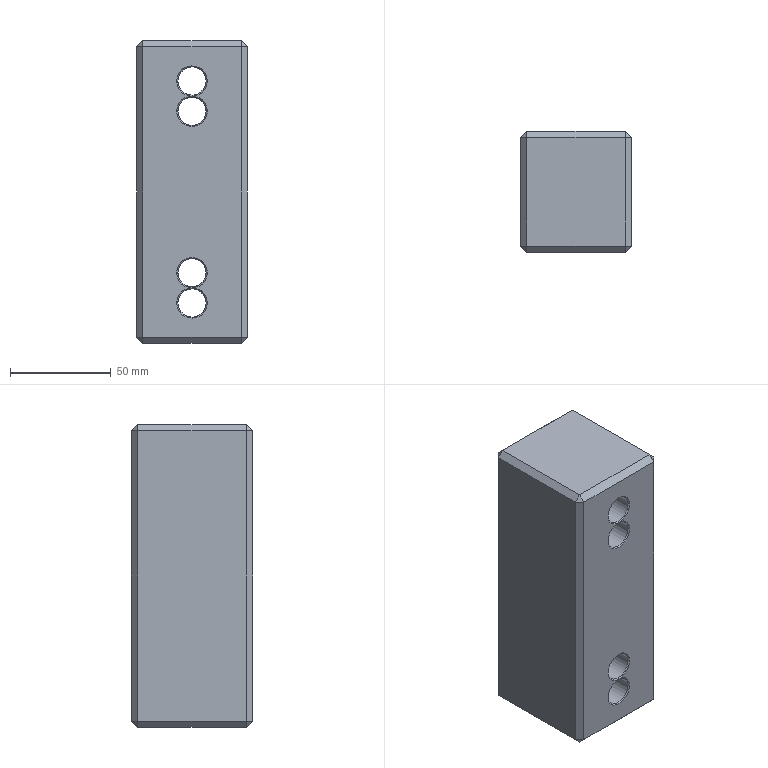Component | NX | SUPPORTING_PLATE | 1 solid | 38 faces | volume 453384 mm3 | plane 26 | cone 8 | cylinder 4 | commonest cylinder face diameters 14 x4